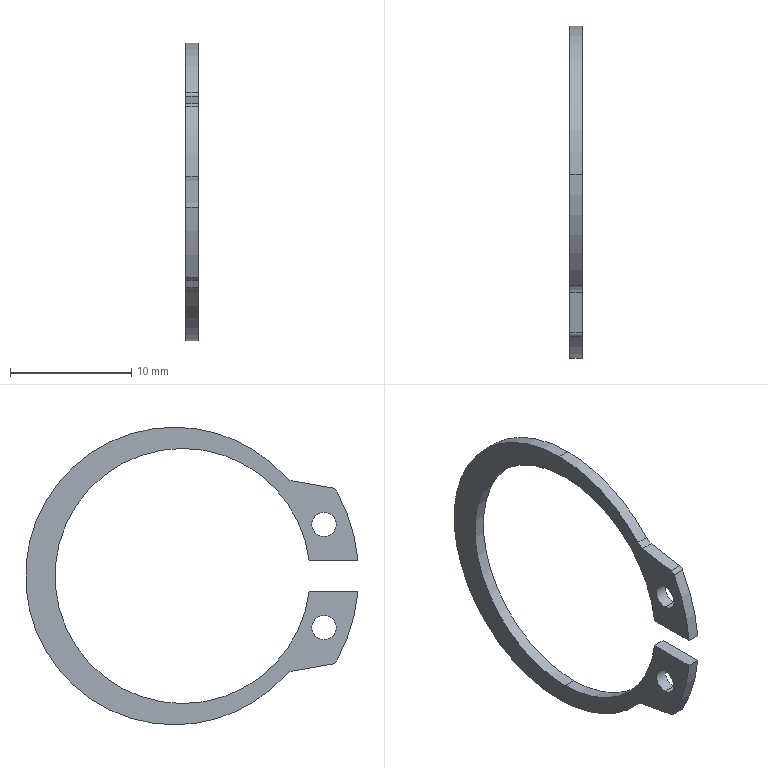Component | SolidWorks | XXXXX08-01-040514RotaryDriveShaft-1_22_T894.1-1 | 1 solid | 22 faces | box 1 x 27.37 x 24.5 mm | volume 155 mm3 | cylinder 16 | plane 6 | commonest cylinder face diameters 2 x6 24.5 x3 21 x3 1 x2 29 x2 | material 65Mn
build123d program:
from build123d import *

# Parameters (mm, degrees)
MATRIX_EXTRUDE_DEPTH      = 0.5
MATRIX_EXTRUDE_DEPTH_BACK = 0.5
SKETCH1_R                 = 1


with BuildPart() as part:
    # Sketch1 → Matrix-Extrude (new, two sides: drawn at the far end of the back side and taken through both)
    with BuildSketch(Plane.XY.offset(-MATRIX_EXTRUDE_DEPTH_BACK)):
        with BuildLine():
            Line((-1.25, -11.095), (-1.25, -15.116))
            ThreePointArc((-1.25, -15.116), (-4.216, -14.544), (-6.999, -13.369))
            ThreePointArc((-6.999, -13.369), (-7.164, -13.222), (-7.25, -13.018))
            Line((-7.25, -13.018), (-7.832, -9.717))
            ThreePointArc((-7.832, -9.717), (-7.943, -9.404), (-8.151, -9.144))
            ThreePointArc((-8.151, -9.144), (0, 12.25), (8.151, -9.144))
            ThreePointArc((8.151, -9.144), (7.943, -9.404), (7.832, -9.717))
            Line((7.832, -9.717), (7.25, -13.018))
            ThreePointArc((7.25, -13.018), (7.164, -13.222), (6.999, -13.369))
            ThreePointArc((6.999, -13.369), (4.216, -14.544), (1.25, -15.116))
            Line((1.25, -15.116), (1.25, -11.095))
            ThreePointArc((1.25, -11.095), (0, 9.83), (-1.25, -11.095))
        make_face()
        with Locations((-4.25, -12.319)):
            Circle(SKETCH1_R, mode=Mode.SUBTRACT)
        with Locations(Location((4.25, -12.319, 0), (0, 0, 180))):
            Circle(SKETCH1_R, mode=Mode.SUBTRACT)
    extrude(amount=MATRIX_EXTRUDE_DEPTH + MATRIX_EXTRUDE_DEPTH_BACK)


solid = part.part

# Placed as in the assembly
solid = solid.moved(Location((-29.2, 0.67, 0), (0, 90, 0)))
STEP:
#1=CARTESIAN_POINT('',(-1.13,-0.4586,-0.128));
#2=VERTEX_POINT('',#1);
#3=CARTESIAN_POINT('',(-1.13,-0.4586,-0.2067));
#4=VERTEX_POINT('',#3);
#5=CARTESIAN_POINT('',(-1.13,-0.4586,-0.1673));
#6=DIRECTION('',(1.,0.,0.));
#7=DIRECTION('',(0.,0.,1.));
#8=AXIS2_PLACEMENT_3D('',#5,#6,#7);
#9=CIRCLE('',#8,0.03937);
#10=EDGE_CURVE('',#2,#4,#9,.T.);
#11=ORIENTED_EDGE('',*,*,#10,.T.);
#12=CARTESIAN_POINT('',(-1.169,-0.4586,-0.2067));
#13=VERTEX_POINT('',#12);
#14=CARTESIAN_POINT('',(-1.13,-0.4586,-0.2067));
#15=DIRECTION('',(-1.,0.,0.));
#16=VECTOR('',#15,39.37);
#17=LINE('',#14,#16);
#18=EDGE_CURVE('',#4,#13,#17,.T.);
#19=ORIENTED_EDGE('',*,*,#18,.T.);
#20=CARTESIAN_POINT('',(-1.169,-0.4586,-0.128));
#21=VERTEX_POINT('',#20);
#22=CARTESIAN_POINT('',(-1.169,-0.4586,-0.1673));
#23=DIRECTION('',(1.,0.,0.));
#24=DIRECTION('',(0.,0.,1.));
#25=AXIS2_PLACEMENT_3D('',#22,#23,#24);
#26=CIRCLE('',#25,0.03937);
#27=EDGE_CURVE('',#21,#13,#26,.T.);
#28=ORIENTED_EDGE('',*,*,#27,.F.);
#29=CARTESIAN_POINT('',(-1.13,-0.4586,-0.128));
#30=DIRECTION('',(-1.,0.,0.));
#31=VECTOR('',#30,39.37);
#32=LINE('',#29,#31);
#33=EDGE_CURVE('',#2,#21,#32,.T.);
#34=ORIENTED_EDGE('',*,*,#33,.F.);
#35=EDGE_LOOP('',(#11,#19,#28,#34));
#36=FACE_OUTER_BOUND('',#35,.T.);
#37=CARTESIAN_POINT('',(-1.13,-0.4586,-0.1673));
#38=DIRECTION('',(-1.,0.,0.));
#39=DIRECTION('',(0.,0.,1.));
#40=AXIS2_PLACEMENT_3D('',#37,#38,#39);
#41=CYLINDRICAL_SURFACE('',#40,0.03937);
#42=ADVANCED_FACE('',(#36),#41,.F.);
#43=CARTESIAN_POINT('',(-1.13,-0.4586,0.2067));
#44=VERTEX_POINT('',#43);
#45=CARTESIAN_POINT('',(-1.13,-0.4586,0.128));
#46=VERTEX_POINT('',#45);
#47=CARTESIAN_POINT('',(-1.13,-0.4586,0.1673));
#48=DIRECTION('',(1.,0.,0.));
#49=DIRECTION('',(0.,0.,-1.));
#50=AXIS2_PLACEMENT_3D('',#47,#48,#49);
#51=CIRCLE('',#50,0.03937);
#52=EDGE_CURVE('',#44,#46,#51,.T.);
#53=ORIENTED_EDGE('',*,*,#52,.T.);
#54=CARTESIAN_POINT('',(-1.169,-0.4586,0.128));
#55=VERTEX_POINT('',#54);
#56=CARTESIAN_POINT('',(-1.13,-0.4586,0.128));
#57=DIRECTION('',(-1.,0.,0.));
#58=VECTOR('',#57,39.37);
#59=LINE('',#56,#58);
#60=EDGE_CURVE('',#46,#55,#59,.T.);
#61=ORIENTED_EDGE('',*,*,#60,.T.);
#62=CARTESIAN_POINT('',(-1.169,-0.4586,0.2067));
#63=VERTEX_POINT('',#62);
#64=CARTESIAN_POINT('',(-1.169,-0.4586,0.1673));
#65=DIRECTION('',(1.,0.,0.));
#66=DIRECTION('',(0.,0.,-1.));
#67=AXIS2_PLACEMENT_3D('',#64,#65,#66);
#68=CIRCLE('',#67,0.03937);
#69=EDGE_CURVE('',#63,#55,#68,.T.);
#70=ORIENTED_EDGE('',*,*,#69,.F.);
#71=CARTESIAN_POINT('',(-1.13,-0.4586,0.2067));
#72=DIRECTION('',(-1.,0.,0.));
#73=VECTOR('',#72,39.37);
#74=LINE('',#71,#73);
#75=EDGE_CURVE('',#44,#63,#74,.T.);
#76=ORIENTED_EDGE('',*,*,#75,.F.);
#77=EDGE_LOOP('',(#53,#61,#70,#76));
#78=FACE_OUTER_BOUND('',#77,.T.);
#79=CARTESIAN_POINT('',(-1.13,-0.4586,0.1673));
#80=DIRECTION('',(-1.,0.,0.));
#81=DIRECTION('',(0.,0.,1.));
#82=AXIS2_PLACEMENT_3D('',#79,#80,#81);
#83=CYLINDRICAL_SURFACE('',#82,0.03937);
#84=ADVANCED_FACE('',(#78),#83,.F.);
#85=CARTESIAN_POINT('',(-1.13,0.02638,-0.4823));
#86=VERTEX_POINT('',#85);
#87=CARTESIAN_POINT('',(-1.13,0.02638,0.4823));
#88=VERTEX_POINT('',#87);
#89=CARTESIAN_POINT('',(-1.13,0.02638,-0.));
#90=DIRECTION('',(1.,0.,0.));
#91=DIRECTION('',(0.,0.,-1.));
#92=AXIS2_PLACEMENT_3D('',#89,#90,#91);
#93=CIRCLE('',#92,0.4823);
#94=EDGE_CURVE('',#86,#88,#93,.T.);
#95=ORIENTED_EDGE('',*,*,#94,.F.);
#96=CARTESIAN_POINT('',(-1.169,0.02638,-0.4823));
#97=VERTEX_POINT('',#96);
#98=CARTESIAN_POINT('',(-1.13,0.02638,-0.4823));
#99=DIRECTION('',(-1.,0.,0.));
#100=VECTOR('',#99,39.37);
#101=LINE('',#98,#100);
#102=EDGE_CURVE('',#86,#97,#101,.T.);
#103=ORIENTED_EDGE('',*,*,#102,.T.);
#104=CARTESIAN_POINT('',(-1.169,0.02638,0.4823));
#105=VERTEX_POINT('',#104);
#106=CARTESIAN_POINT('',(-1.169,0.02638,-0.));
#107=DIRECTION('',(1.,0.,0.));
#108=DIRECTION('',(0.,0.,-1.));
#109=AXIS2_PLACEMENT_3D('',#106,#107,#108);
#110=CIRCLE('',#109,0.4823);
#111=EDGE_CURVE('',#97,#105,#110,.T.);
#112=ORIENTED_EDGE('',*,*,#111,.T.);
#113=CARTESIAN_POINT('',(-1.13,0.02638,0.4823));
#114=DIRECTION('',(-1.,0.,0.));
#115=VECTOR('',#114,39.37);
#116=LINE('',#113,#115);
#117=EDGE_CURVE('',#88,#105,#116,.T.);
#118=ORIENTED_EDGE('',*,*,#117,.F.);
#119=EDGE_LOOP('',(#95,#103,#112,#118));
#120=FACE_OUTER_BOUND('',#119,.T.);
#121=CARTESIAN_POINT('',(-1.13,0.02638,-0.));
#122=DIRECTION('',(-1.,0.,0.));
#123=DIRECTION('',(0.,0.,1.));
#124=AXIS2_PLACEMENT_3D('',#121,#122,#123);
#125=CYLINDRICAL_SURFACE('',#124,0.4823);
#126=ADVANCED_FACE('',(#120),#125,.T.);
#127=CARTESIAN_POINT('',(-1.13,-0.3336,0.3209));
#128=VERTEX_POINT('',#127);
#129=CARTESIAN_POINT('',(-1.13,0.02638,-0.));
#130=DIRECTION('',(1.,0.,0.));
#131=DIRECTION('',(0.,0.,-1.));
#132=AXIS2_PLACEMENT_3D('',#129,#130,#131);
#133=CIRCLE('',#132,0.4823);
#134=EDGE_CURVE('',#88,#128,#133,.T.);
#135=ORIENTED_EDGE('',*,*,#134,.F.);
#136=ORIENTED_EDGE('',*,*,#117,.T.);
#137=CARTESIAN_POINT('',(-1.169,-0.3336,0.3209));
#138=VERTEX_POINT('',#137);
#139=CARTESIAN_POINT('',(-1.169,0.02638,-0.));
#140=DIRECTION('',(1.,0.,0.));
#141=DIRECTION('',(0.,0.,-1.));
#142=AXIS2_PLACEMENT_3D('',#139,#140,#141);
#143=CIRCLE('',#142,0.4823);
#144=EDGE_CURVE('',#105,#138,#143,.T.);
#145=ORIENTED_EDGE('',*,*,#144,.T.);
#146=CARTESIAN_POINT('',(-1.13,-0.3336,0.3209));
#147=DIRECTION('',(-1.,0.,0.));
#148=VECTOR('',#147,39.37);
#149=LINE('',#146,#148);
#150=EDGE_CURVE('',#128,#138,#149,.T.);
#151=ORIENTED_EDGE('',*,*,#150,.F.);
#152=EDGE_LOOP('',(#135,#136,#145,#151));
#153=FACE_OUTER_BOUND('',#152,.T.);
#154=CARTESIAN_POINT('',(-1.13,0.02638,-0.));
#155=DIRECTION('',(-1.,0.,0.));
#156=DIRECTION('',(0.,0.,1.));
#157=AXIS2_PLACEMENT_3D('',#154,#155,#156);
#158=CYLINDRICAL_SURFACE('',#157,0.4823);
#159=ADVANCED_FACE('',(#153),#158,.T.);
#160=CARTESIAN_POINT('',(-1.13,0.,-0.4134));
#161=VERTEX_POINT('',#160);
#162=CARTESIAN_POINT('',(-1.13,-0.4104,-0.04921));
#163=VERTEX_POINT('',#162);
#164=CARTESIAN_POINT('',(-1.13,0.,-0.));
#165=DIRECTION('',(-1.,0.,0.));
#166=DIRECTION('',(0.,0.,-1.));
#167=AXIS2_PLACEMENT_3D('',#164,#165,#166);
#168=CIRCLE('',#167,0.4134);
#169=EDGE_CURVE('',#161,#163,#168,.T.);
#170=ORIENTED_EDGE('',*,*,#169,.F.);
#171=CARTESIAN_POINT('',(-1.169,0.,-0.4134));
#172=VERTEX_POINT('',#171);
#173=CARTESIAN_POINT('',(-1.13,0.,-0.4134));
#174=DIRECTION('',(-1.,0.,0.));
#175=VECTOR('',#174,39.37);
#176=LINE('',#173,#175);
#177=EDGE_CURVE('',#161,#172,#176,.T.);
#178=ORIENTED_EDGE('',*,*,#177,.T.);
#179=CARTESIAN_POINT('',(-1.169,-0.4104,-0.04921));
#180=VERTEX_POINT('',#179);
#181=CARTESIAN_POINT('',(-1.169,0.,-0.));
#182=DIRECTION('',(-1.,0.,0.));
#183=DIRECTION('',(0.,0.,-1.));
#184=AXIS2_PLACEMENT_3D('',#181,#182,#183);
#185=CIRCLE('',#184,0.4134);
#186=EDGE_CURVE('',#172,#180,#185,.T.);
#187=ORIENTED_EDGE('',*,*,#186,.T.);
#188=CARTESIAN_POINT('',(-1.13,-0.4104,-0.04921));
#189=DIRECTION('',(-1.,0.,0.));
#190=VECTOR('',#189,39.37);
#191=LINE('',#188,#190);
#192=EDGE_CURVE('',#163,#180,#191,.T.);
#193=ORIENTED_EDGE('',*,*,#192,.F.);
#194=EDGE_LOOP('',(#170,#178,#187,#193));
#195=FACE_OUTER_BOUND('',#194,.T.);
#196=CARTESIAN_POINT('',(-1.13,0.,-0.));
#197=DIRECTION('',(-1.,0.,0.));
#198=DIRECTION('',(0.,0.,1.));
#199=AXIS2_PLACEMENT_3D('',#196,#197,#198);
#200=CYLINDRICAL_SURFACE('',#199,0.4134);
#201=ADVANCED_FACE('',(#195),#200,.F.);
#202=ORIENTED_EDGE('',*,*,#177,.F.);
#203=CARTESIAN_POINT('',(-1.13,0.,0.4134));
#204=VERTEX_POINT('',#203);
#205=CARTESIAN_POINT('',(-1.13,0.,-0.));
#206=DIRECTION('',(-1.,0.,0.));
#207=DIRECTION('',(0.,0.,-1.));
#208=AXIS2_PLACEMENT_3D('',#205,#206,#207);
#209=CIRCLE('',#208,0.4134);
#210=EDGE_CURVE('',#204,#161,#209,.T.);
#211=ORIENTED_EDGE('',*,*,#210,.F.);
#212=CARTESIAN_POINT('',(-1.169,0.,0.4134));
#213=VERTEX_POINT('',#212);
#214=CARTESIAN_POINT('',(-1.13,0.,0.4134));
#215=DIRECTION('',(-1.,0.,0.));
#216=VECTOR('',#215,39.37);
#217=LINE('',#214,#216);
#218=EDGE_CURVE('',#204,#213,#217,.T.);
#219=ORIENTED_EDGE('',*,*,#218,.T.);
#220=CARTESIAN_POINT('',(-1.169,0.,-0.));
#221=DIRECTION('',(-1.,0.,0.));
#222=DIRECTION('',(0.,0.,-1.));
#223=AXIS2_PLACEMENT_3D('',#220,#221,#222);
#224=CIRCLE('',#223,0.4134);
#225=EDGE_CURVE('',#213,#172,#224,.T.);
#226=ORIENTED_EDGE('',*,*,#225,.T.);
#227=EDGE_LOOP('',(#202,#211,#219,#226));
#228=FACE_OUTER_BOUND('',#227,.T.);
#229=CARTESIAN_POINT('',(-1.13,0.,-0.));
#230=DIRECTION('',(-1.,0.,0.));
#231=DIRECTION('',(0.,0.,1.));
#232=AXIS2_PLACEMENT_3D('',#229,#230,#231);
#233=CYLINDRICAL_SURFACE('',#232,0.4134);
#234=ADVANCED_FACE('',(#228),#233,.F.);
#235=ORIENTED_EDGE('',*,*,#52,.F.);
#236=CARTESIAN_POINT('',(-1.13,-0.4586,0.1673));
#237=DIRECTION('',(1.,0.,0.));
#238=DIRECTION('',(0.,0.,-1.));
#239=AXIS2_PLACEMENT_3D('',#236,#237,#238);
#240=CIRCLE('',#239,0.03937);
#241=EDGE_CURVE('',#46,#44,#240,.T.);
#242=ORIENTED_EDGE('',*,*,#241,.F.);
#243=EDGE_LOOP('',(#235,#242));
#244=FACE_BOUND('',#243,.T.);
#245=CARTESIAN_POINT('',(-1.13,-0.3562,0.3083));
#246=VERTEX_POINT('',#245);
#247=CARTESIAN_POINT('',(-1.13,-0.363,0.3471));
#248=DIRECTION('',(-1.,0.,0.));
#249=DIRECTION('',(0.,0.,-1.));
#250=AXIS2_PLACEMENT_3D('',#247,#248,#249);
#251=CIRCLE('',#250,0.03937);
#252=EDGE_CURVE('',#128,#246,#251,.T.);
#253=ORIENTED_EDGE('',*,*,#252,.T.);
#254=CARTESIAN_POINT('',(-1.13,-0.4861,0.2854));
#255=VERTEX_POINT('',#254);
#256=CARTESIAN_POINT('',(-1.13,-0.3562,0.3083));
#257=DIRECTION('',(0.,-0.9848,-0.1736));
#258=VECTOR('',#257,39.37);
#259=LINE('',#256,#258);
#260=EDGE_CURVE('',#246,#255,#259,.T.);
#261=ORIENTED_EDGE('',*,*,#260,.T.);
#262=CARTESIAN_POINT('',(-1.13,-0.5,0.2755));
#263=VERTEX_POINT('',#262);
#264=CARTESIAN_POINT('',(-1.13,-0.4827,0.266));
#265=DIRECTION('',(1.,0.,0.));
#266=DIRECTION('',(0.,0.,1.));
#267=AXIS2_PLACEMENT_3D('',#264,#265,#266);
#268=CIRCLE('',#267,0.01969);
#269=EDGE_CURVE('',#255,#263,#268,.T.);
#270=ORIENTED_EDGE('',*,*,#269,.T.);
#271=CARTESIAN_POINT('',(-1.13,-0.5687,0.04921));
#272=VERTEX_POINT('',#271);
#273=CARTESIAN_POINT('',(-1.13,0.,-0.));
#274=DIRECTION('',(1.,0.,0.));
#275=DIRECTION('',(0.,0.,1.));
#276=AXIS2_PLACEMENT_3D('',#273,#274,#275);
#277=CIRCLE('',#276,0.5709);
#278=EDGE_CURVE('',#263,#272,#277,.T.);
#279=ORIENTED_EDGE('',*,*,#278,.T.);
#280=CARTESIAN_POINT('',(-1.13,-0.4104,0.04921));
#281=VERTEX_POINT('',#280);
#282=CARTESIAN_POINT('',(-1.13,-0.4104,0.04921));
#283=DIRECTION('',(0.,1.,0.));
#284=VECTOR('',#283,39.37);
#285=LINE('',#282,#284);
#286=EDGE_CURVE('',#272,#281,#285,.T.);
#287=ORIENTED_EDGE('',*,*,#286,.T.);
#288=CARTESIAN_POINT('',(-1.13,0.,-0.));
#289=DIRECTION('',(-1.,0.,0.));
#290=DIRECTION('',(0.,0.,-1.));
#291=AXIS2_PLACEMENT_3D('',#288,#289,#290);
#292=CIRCLE('',#291,0.4134);
#293=EDGE_CURVE('',#281,#204,#292,.T.);
#294=ORIENTED_EDGE('',*,*,#293,.T.);
#295=ORIENTED_EDGE('',*,*,#210,.T.);
#296=ORIENTED_EDGE('',*,*,#169,.T.);
#297=CARTESIAN_POINT('',(-1.13,-0.5687,-0.04921));
#298=VERTEX_POINT('',#297);
#299=CARTESIAN_POINT('',(-1.13,-0.4104,-0.04921));
#300=DIRECTION('',(0.,-1.,-0.));
#301=VECTOR('',#300,39.37);
#302=LINE('',#299,#301);
#303=EDGE_CURVE('',#163,#298,#302,.T.);
#304=ORIENTED_EDGE('',*,*,#303,.T.);
#305=CARTESIAN_POINT('',(-1.13,-0.5,-0.2755));
#306=VERTEX_POINT('',#305);
#307=CARTESIAN_POINT('',(-1.13,0.,-0.));
#308=DIRECTION('',(1.,0.,0.));
#309=DIRECTION('',(0.,0.,-1.));
#310=AXIS2_PLACEMENT_3D('',#307,#308,#309);
#311=CIRCLE('',#310,0.5709);
#312=EDGE_CURVE('',#298,#306,#311,.T.);
#313=ORIENTED_EDGE('',*,*,#312,.T.);
#314=CARTESIAN_POINT('',(-1.13,-0.4861,-0.2854));
#315=VERTEX_POINT('',#314);
#316=CARTESIAN_POINT('',(-1.13,-0.4827,-0.266));
#317=DIRECTION('',(1.,0.,0.));
#318=DIRECTION('',(0.,0.,-1.));
#319=AXIS2_PLACEMENT_3D('',#316,#317,#318);
#320=CIRCLE('',#319,0.01969);
#321=EDGE_CURVE('',#306,#315,#320,.T.);
#322=ORIENTED_EDGE('',*,*,#321,.T.);
#323=CARTESIAN_POINT('',(-1.13,-0.3562,-0.3083));
#324=VERTEX_POINT('',#323);
#325=CARTESIAN_POINT('',(-1.13,-0.3562,-0.3083));
#326=DIRECTION('',(0.,0.9848,-0.1736));
#327=VECTOR('',#326,39.37);
#328=LINE('',#325,#327);
#329=EDGE_CURVE('',#315,#324,#328,.T.);
#330=ORIENTED_EDGE('',*,*,#329,.T.);
#331=CARTESIAN_POINT('',(-1.13,-0.3336,-0.3209));
#332=VERTEX_POINT('',#331);
#333=CARTESIAN_POINT('',(-1.13,-0.363,-0.3471));
#334=DIRECTION('',(-1.,0.,0.));
#335=DIRECTION('',(0.,0.,1.));
#336=AXIS2_PLACEMENT_3D('',#333,#334,#335);
#337=CIRCLE('',#336,0.03937);
#338=EDGE_CURVE('',#324,#332,#337,.T.);
#339=ORIENTED_EDGE('',*,*,#338,.T.);
#340=CARTESIAN_POINT('',(-1.13,0.02638,-0.));
#341=DIRECTION('',(1.,0.,0.));
#342=DIRECTION('',(0.,0.,-1.));
#343=AXIS2_PLACEMENT_3D('',#340,#341,#342);
#344=CIRCLE('',#343,0.4823);
#345=EDGE_CURVE('',#332,#86,#344,.T.);
#346=ORIENTED_EDGE('',*,*,#345,.T.);
#347=ORIENTED_EDGE('',*,*,#94,.T.);
#348=ORIENTED_EDGE('',*,*,#134,.T.);
#349=EDGE_LOOP('',(#253,#261,#270,#279,#287,#294,#295,#296,#304,#313,#322,#330,#339,#346,#347,#348));
#350=FACE_OUTER_BOUND('',#349,.T.);
#351=ORIENTED_EDGE('',*,*,#10,.F.);
#352=CARTESIAN_POINT('',(-1.13,-0.4586,-0.1673));
#353=DIRECTION('',(1.,0.,0.));
#354=DIRECTION('',(0.,0.,1.));
#355=AXIS2_PLACEMENT_3D('',#352,#353,#354);
#356=CIRCLE('',#355,0.03937);
#357=EDGE_CURVE('',#4,#2,#356,.T.);
#358=ORIENTED_EDGE('',*,*,#357,.F.);
#359=EDGE_LOOP('',(#351,#358));
#360=FACE_BOUND('',#359,.T.);
#361=CARTESIAN_POINT('',(-1.13,-0.363,0.3471));
#362=DIRECTION('',(1.,0.,0.));
#363=DIRECTION('',(0.,0.,-1.));
#364=AXIS2_PLACEMENT_3D('',#361,#362,#363);
#365=PLANE('',#364);
#366=ADVANCED_FACE('',(#244,#350,#360),#365,.T.);
#367=ORIENTED_EDGE('',*,*,#150,.T.);
#368=CARTESIAN_POINT('',(-1.169,-0.3562,0.3083));
#369=VERTEX_POINT('',#368);
#370=CARTESIAN_POINT('',(-1.169,-0.363,0.3471));
#371=DIRECTION('',(-1.,0.,0.));
#372=DIRECTION('',(0.,0.,-1.));
#373=AXIS2_PLACEMENT_3D('',#370,#371,#372);
#374=CIRCLE('',#373,0.03937);
#375=EDGE_CURVE('',#138,#369,#374,.T.);
#376=ORIENTED_EDGE('',*,*,#375,.T.);
#377=CARTESIAN_POINT('',(-1.13,-0.3562,0.3083));
#378=DIRECTION('',(-1.,0.,0.));
#379=VECTOR('',#378,39.37);
#380=LINE('',#377,#379);
#381=EDGE_CURVE('',#246,#369,#380,.T.);
#382=ORIENTED_EDGE('',*,*,#381,.F.);
#383=ORIENTED_EDGE('',*,*,#252,.F.);
#384=EDGE_LOOP('',(#367,#376,#382,#383));
#385=FACE_OUTER_BOUND('',#384,.T.);
#386=CARTESIAN_POINT('',(-1.13,-0.363,0.3471));
#387=DIRECTION('',(-1.,0.,0.));
#388=DIRECTION('',(0.,0.,1.));
#389=AXIS2_PLACEMENT_3D('',#386,#387,#388);
#390=CYLINDRICAL_SURFACE('',#389,0.03937);
#391=ADVANCED_FACE('',(#385),#390,.F.);
#392=ORIENTED_EDGE('',*,*,#381,.T.);
#393=CARTESIAN_POINT('',(-1.169,-0.4861,0.2854));
#394=VERTEX_POINT('',#393);
#395=CARTESIAN_POINT('',(-1.169,-0.3562,0.3083));
#396=DIRECTION('',(0.,-0.9848,-0.1736));
#397=VECTOR('',#396,39.37);
#398=LINE('',#395,#397);
#399=EDGE_CURVE('',#369,#394,#398,.T.);
#400=ORIENTED_EDGE('',*,*,#399,.T.);
#401=CARTESIAN_POINT('',(-1.13,-0.4861,0.2854));
#402=DIRECTION('',(-1.,0.,0.));
#403=VECTOR('',#402,39.37);
#404=LINE('',#401,#403);
#405=EDGE_CURVE('',#255,#394,#404,.T.);
#406=ORIENTED_EDGE('',*,*,#405,.F.);
#407=ORIENTED_EDGE('',*,*,#260,.F.);
#408=EDGE_LOOP('',(#392,#400,#406,#407));
#409=FACE_OUTER_BOUND('',#408,.T.);
#410=CARTESIAN_POINT('',(-1.13,-0.3562,0.3083));
#411=DIRECTION('',(0.,0.1736,-0.9848));
#412=DIRECTION('',(0.,0.9848,0.1736));
#413=AXIS2_PLACEMENT_3D('',#410,#411,#412);
#414=PLANE('',#413);
#415=ADVANCED_FACE('',(#409),#414,.F.);
#416=ORIENTED_EDGE('',*,*,#405,.T.);
#417=CARTESIAN_POINT('',(-1.169,-0.5,0.2755));
#418=VERTEX_POINT('',#417);
#419=CARTESIAN_POINT('',(-1.169,-0.4827,0.266));
#420=DIRECTION('',(1.,0.,0.));
#421=DIRECTION('',(0.,0.,1.));
#422=AXIS2_PLACEMENT_3D('',#419,#420,#421);
#423=CIRCLE('',#422,0.01969);
#424=EDGE_CURVE('',#394,#418,#423,.T.);
#425=ORIENTED_EDGE('',*,*,#424,.T.);
#426=CARTESIAN_POINT('',(-1.13,-0.5,0.2755));
#427=DIRECTION('',(-1.,0.,0.));
#428=VECTOR('',#427,39.37);
#429=LINE('',#426,#428);
#430=EDGE_CURVE('',#263,#418,#429,.T.);
#431=ORIENTED_EDGE('',*,*,#430,.F.);
#432=ORIENTED_EDGE('',*,*,#269,.F.);
#433=EDGE_LOOP('',(#416,#425,#431,#432));
#434=FACE_OUTER_BOUND('',#433,.T.);
#435=CARTESIAN_POINT('',(-1.13,-0.4827,0.266));
#436=DIRECTION('',(-1.,0.,0.));
#437=DIRECTION('',(0.,0.,1.));
#438=AXIS2_PLACEMENT_3D('',#435,#436,#437);
#439=CYLINDRICAL_SURFACE('',#438,0.01969);
#440=ADVANCED_FACE('',(#434),#439,.T.);
#441=ORIENTED_EDGE('',*,*,#430,.T.);
#442=CARTESIAN_POINT('',(-1.169,-0.5687,0.04921));
#443=VERTEX_POINT('',#442);
#444=CARTESIAN_POINT('',(-1.169,0.,-0.));
#445=DIRECTION('',(1.,0.,0.));
#446=DIRECTION('',(0.,0.,1.));
#447=AXIS2_PLACEMENT_3D('',#444,#445,#446);
#448=CIRCLE('',#447,0.5709);
#449=EDGE_CURVE('',#418,#443,#448,.T.);
#450=ORIENTED_EDGE('',*,*,#449,.T.);
#451=CARTESIAN_POINT('',(-1.13,-0.5687,0.04921));
#452=DIRECTION('',(-1.,0.,0.));
#453=VECTOR('',#452,39.37);
#454=LINE('',#451,#453);
#455=EDGE_CURVE('',#272,#443,#454,.T.);
#456=ORIENTED_EDGE('',*,*,#455,.F.);
#457=ORIENTED_EDGE('',*,*,#278,.F.);
#458=EDGE_LOOP('',(#441,#450,#456,#457));
#459=FACE_OUTER_BOUND('',#458,.T.);
#460=CARTESIAN_POINT('',(-1.13,0.,-0.));
#461=DIRECTION('',(-1.,0.,0.));
#462=DIRECTION('',(0.,0.,1.));
#463=AXIS2_PLACEMENT_3D('',#460,#461,#462);
#464=CYLINDRICAL_SURFACE('',#463,0.5709);
#465=ADVANCED_FACE('',(#459),#464,.T.);
#466=ORIENTED_EDGE('',*,*,#455,.T.);
#467=CARTESIAN_POINT('',(-1.169,-0.4104,0.04921));
#468=VERTEX_POINT('',#467);
#469=CARTESIAN_POINT('',(-1.169,-0.4104,0.04921));
#470=DIRECTION('',(0.,1.,0.));
#471=VECTOR('',#470,39.37);
#472=LINE('',#469,#471);
#473=EDGE_CURVE('',#443,#468,#472,.T.);
#474=ORIENTED_EDGE('',*,*,#473,.T.);
#475=CARTESIAN_POINT('',(-1.13,-0.4104,0.04921));
#476=DIRECTION('',(-1.,0.,0.));
#477=VECTOR('',#476,39.37);
#478=LINE('',#475,#477);
#479=EDGE_CURVE('',#281,#468,#478,.T.);
#480=ORIENTED_EDGE('',*,*,#479,.F.);
#481=ORIENTED_EDGE('',*,*,#286,.F.);
#482=EDGE_LOOP('',(#466,#474,#480,#481));
#483=FACE_OUTER_BOUND('',#482,.T.);
#484=CARTESIAN_POINT('',(-1.13,-0.4104,0.04921));
#485=DIRECTION('',(0.,-0.,1.));
#486=DIRECTION('',(0.,-1.,-0.));
#487=AXIS2_PLACEMENT_3D('',#484,#485,#486);
#488=PLANE('',#487);
#489=ADVANCED_FACE('',(#483),#488,.F.);
#490=ORIENTED_EDGE('',*,*,#218,.F.);
#491=ORIENTED_EDGE('',*,*,#293,.F.);
#492=ORIENTED_EDGE('',*,*,#479,.T.);
#493=CARTESIAN_POINT('',(-1.169,0.,-0.));
#494=DIRECTION('',(-1.,0.,0.));
#495=DIRECTION('',(0.,0.,-1.));
#496=AXIS2_PLACEMENT_3D('',#493,#494,#495);
#497=CIRCLE('',#496,0.4134);
#498=EDGE_CURVE('',#468,#213,#497,.T.);
#499=ORIENTED_EDGE('',*,*,#498,.T.);
#500=EDGE_LOOP('',(#490,#491,#492,#499));
#501=FACE_OUTER_BOUND('',#500,.T.);
#502=CARTESIAN_POINT('',(-1.13,0.,-0.));
#503=DIRECTION('',(-1.,0.,0.));
#504=DIRECTION('',(0.,0.,1.));
#505=AXIS2_PLACEMENT_3D('',#502,#503,#504);
#506=CYLINDRICAL_SURFACE('',#505,0.4134);
#507=ADVANCED_FACE('',(#501),#506,.F.);
#508=ORIENTED_EDGE('',*,*,#192,.T.);
#509=CARTESIAN_POINT('',(-1.169,-0.5687,-0.04921));
#510=VERTEX_POINT('',#509);
#511=CARTESIAN_POINT('',(-1.169,-0.4104,-0.04921));
#512=DIRECTION('',(0.,-1.,-0.));
#513=VECTOR('',#512,39.37);
#514=LINE('',#511,#513);
#515=EDGE_CURVE('',#180,#510,#514,.T.);
#516=ORIENTED_EDGE('',*,*,#515,.T.);
#517=CARTESIAN_POINT('',(-1.13,-0.5687,-0.04921));
#518=DIRECTION('',(-1.,0.,0.));
#519=VECTOR('',#518,39.37);
#520=LINE('',#517,#519);
#521=EDGE_CURVE('',#298,#510,#520,.T.);
#522=ORIENTED_EDGE('',*,*,#521,.F.);
#523=ORIENTED_EDGE('',*,*,#303,.F.);
#524=EDGE_LOOP('',(#508,#516,#522,#523));
#525=FACE_OUTER_BOUND('',#524,.T.);
#526=CARTESIAN_POINT('',(-1.13,-0.4104,-0.04921));
#527=DIRECTION('',(0.,0.,-1.));
#528=DIRECTION('',(0.,1.,0.));
#529=AXIS2_PLACEMENT_3D('',#526,#527,#528);
#530=PLANE('',#529);
#531=ADVANCED_FACE('',(#525),#530,.F.);
#532=ORIENTED_EDGE('',*,*,#521,.T.);
#533=CARTESIAN_POINT('',(-1.169,-0.5,-0.2755));
#534=VERTEX_POINT('',#533);
#535=CARTESIAN_POINT('',(-1.169,0.,-0.));
#536=DIRECTION('',(1.,0.,0.));
#537=DIRECTION('',(0.,0.,-1.));
#538=AXIS2_PLACEMENT_3D('',#535,#536,#537);
#539=CIRCLE('',#538,0.5709);
#540=EDGE_CURVE('',#510,#534,#539,.T.);
#541=ORIENTED_EDGE('',*,*,#540,.T.);
#542=CARTESIAN_POINT('',(-1.13,-0.5,-0.2755));
#543=DIRECTION('',(-1.,0.,0.));
#544=VECTOR('',#543,39.37);
#545=LINE('',#542,#544);
#546=EDGE_CURVE('',#306,#534,#545,.T.);
#547=ORIENTED_EDGE('',*,*,#546,.F.);
#548=ORIENTED_EDGE('',*,*,#312,.F.);
#549=EDGE_LOOP('',(#532,#541,#547,#548));
#550=FACE_OUTER_BOUND('',#549,.T.);
#551=CARTESIAN_POINT('',(-1.13,0.,-0.));
#552=DIRECTION('',(-1.,0.,0.));
#553=DIRECTION('',(0.,0.,1.));
#554=AXIS2_PLACEMENT_3D('',#551,#552,#553);
#555=CYLINDRICAL_SURFACE('',#554,0.5709);
#556=ADVANCED_FACE('',(#550),#555,.T.);
#557=ORIENTED_EDGE('',*,*,#546,.T.);
#558=CARTESIAN_POINT('',(-1.169,-0.4861,-0.2854));
#559=VERTEX_POINT('',#558);
#560=CARTESIAN_POINT('',(-1.169,-0.4827,-0.266));
#561=DIRECTION('',(1.,0.,0.));
#562=DIRECTION('',(0.,0.,-1.));
#563=AXIS2_PLACEMENT_3D('',#560,#561,#562);
#564=CIRCLE('',#563,0.01969);
#565=EDGE_CURVE('',#534,#559,#564,.T.);
#566=ORIENTED_EDGE('',*,*,#565,.T.);
#567=CARTESIAN_POINT('',(-1.13,-0.4861,-0.2854));
#568=DIRECTION('',(-1.,0.,0.));
#569=VECTOR('',#568,39.37);
#570=LINE('',#567,#569);
#571=EDGE_CURVE('',#315,#559,#570,.T.);
#572=ORIENTED_EDGE('',*,*,#571,.F.);
#573=ORIENTED_EDGE('',*,*,#321,.F.);
#574=EDGE_LOOP('',(#557,#566,#572,#573));
#575=FACE_OUTER_BOUND('',#574,.T.);
#576=CARTESIAN_POINT('',(-1.13,-0.4827,-0.266));
#577=DIRECTION('',(-1.,0.,0.));
#578=DIRECTION('',(0.,0.,1.));
#579=AXIS2_PLACEMENT_3D('',#576,#577,#578);
#580=CYLINDRICAL_SURFACE('',#579,0.01969);
#581=ADVANCED_FACE('',(#575),#580,.T.);
#582=ORIENTED_EDGE('',*,*,#571,.T.);
#583=CARTESIAN_POINT('',(-1.169,-0.3562,-0.3083));
#584=VERTEX_POINT('',#583);
#585=CARTESIAN_POINT('',(-1.169,-0.3562,-0.3083));
#586=DIRECTION('',(0.,0.9848,-0.1736));
#587=VECTOR('',#586,39.37);
#588=LINE('',#585,#587);
#589=EDGE_CURVE('',#559,#584,#588,.T.);
#590=ORIENTED_EDGE('',*,*,#589,.T.);
#591=CARTESIAN_POINT('',(-1.13,-0.3562,-0.3083));
#592=DIRECTION('',(-1.,0.,0.));
#593=VECTOR('',#592,39.37);
#594=LINE('',#591,#593);
#595=EDGE_CURVE('',#324,#584,#594,.T.);
#596=ORIENTED_EDGE('',*,*,#595,.F.);
#597=ORIENTED_EDGE('',*,*,#329,.F.);
#598=EDGE_LOOP('',(#582,#590,#596,#597));
#599=FACE_OUTER_BOUND('',#598,.T.);
#600=CARTESIAN_POINT('',(-1.13,-0.3562,-0.3083));
#601=DIRECTION('',(0.,0.1736,0.9848));
#602=DIRECTION('',(0.,-0.9848,0.1736));
#603=AXIS2_PLACEMENT_3D('',#600,#601,#602);
#604=PLANE('',#603);
#605=ADVANCED_FACE('',(#599),#604,.F.);
#606=ORIENTED_EDGE('',*,*,#595,.T.);
#607=CARTESIAN_POINT('',(-1.169,-0.3336,-0.3209));
#608=VERTEX_POINT('',#607);
#609=CARTESIAN_POINT('',(-1.169,-0.363,-0.3471));
#610=DIRECTION('',(-1.,0.,0.));
#611=DIRECTION('',(0.,0.,1.));
#612=AXIS2_PLACEMENT_3D('',#609,#610,#611);
#613=CIRCLE('',#612,0.03937);
#614=EDGE_CURVE('',#584,#608,#613,.T.);
#615=ORIENTED_EDGE('',*,*,#614,.T.);
#616=CARTESIAN_POINT('',(-1.13,-0.3336,-0.3209));
#617=DIRECTION('',(-1.,0.,0.));
#618=VECTOR('',#617,39.37);
#619=LINE('',#616,#618);
#620=EDGE_CURVE('',#332,#608,#619,.T.);
#621=ORIENTED_EDGE('',*,*,#620,.F.);
#622=ORIENTED_EDGE('',*,*,#338,.F.);
#623=EDGE_LOOP('',(#606,#615,#621,#622));
#624=FACE_OUTER_BOUND('',#623,.T.);
#625=CARTESIAN_POINT('',(-1.13,-0.363,-0.3471));
#626=DIRECTION('',(-1.,0.,0.));
#627=DIRECTION('',(0.,0.,1.));
#628=AXIS2_PLACEMENT_3D('',#625,#626,#627);
#629=CYLINDRICAL_SURFACE('',#628,0.03937);
#630=ADVANCED_FACE('',(#624),#629,.F.);
#631=ORIENTED_EDGE('',*,*,#102,.F.);
#632=ORIENTED_EDGE('',*,*,#345,.F.);
#633=ORIENTED_EDGE('',*,*,#620,.T.);
#634=CARTESIAN_POINT('',(-1.169,0.02638,-0.));
#635=DIRECTION('',(1.,0.,0.));
#636=DIRECTION('',(0.,0.,-1.));
#637=AXIS2_PLACEMENT_3D('',#634,#635,#636);
#638=CIRCLE('',#637,0.4823);
#639=EDGE_CURVE('',#608,#97,#638,.T.);
#640=ORIENTED_EDGE('',*,*,#639,.T.);
#641=EDGE_LOOP('',(#631,#632,#633,#640));
#642=FACE_OUTER_BOUND('',#641,.T.);
#643=CARTESIAN_POINT('',(-1.13,0.02638,-0.));
#644=DIRECTION('',(-1.,0.,0.));
#645=DIRECTION('',(0.,0.,1.));
#646=AXIS2_PLACEMENT_3D('',#643,#644,#645);
#647=CYLINDRICAL_SURFACE('',#646,0.4823);
#648=ADVANCED_FACE('',(#642),#647,.T.);
#649=ORIENTED_EDGE('',*,*,#60,.F.);
#650=ORIENTED_EDGE('',*,*,#241,.T.);
#651=ORIENTED_EDGE('',*,*,#75,.T.);
#652=CARTESIAN_POINT('',(-1.169,-0.4586,0.1673));
#653=DIRECTION('',(1.,0.,0.));
#654=DIRECTION('',(0.,0.,-1.));
#655=AXIS2_PLACEMENT_3D('',#652,#653,#654);
#656=CIRCLE('',#655,0.03937);
#657=EDGE_CURVE('',#55,#63,#656,.T.);
#658=ORIENTED_EDGE('',*,*,#657,.F.);
#659=EDGE_LOOP('',(#649,#650,#651,#658));
#660=FACE_OUTER_BOUND('',#659,.T.);
#661=CARTESIAN_POINT('',(-1.13,-0.4586,0.1673));
#662=DIRECTION('',(-1.,0.,0.));
#663=DIRECTION('',(0.,0.,1.));
#664=AXIS2_PLACEMENT_3D('',#661,#662,#663);
#665=CYLINDRICAL_SURFACE('',#664,0.03937);
#666=ADVANCED_FACE('',(#660),#665,.F.);
#667=ORIENTED_EDGE('',*,*,#18,.F.);
#668=ORIENTED_EDGE('',*,*,#357,.T.);
#669=ORIENTED_EDGE('',*,*,#33,.T.);
#670=CARTESIAN_POINT('',(-1.169,-0.4586,-0.1673));
#671=DIRECTION('',(1.,0.,0.));
#672=DIRECTION('',(0.,0.,1.));
#673=AXIS2_PLACEMENT_3D('',#670,#671,#672);
#674=CIRCLE('',#673,0.03937);
#675=EDGE_CURVE('',#13,#21,#674,.T.);
#676=ORIENTED_EDGE('',*,*,#675,.F.);
#677=EDGE_LOOP('',(#667,#668,#669,#676));
#678=FACE_OUTER_BOUND('',#677,.T.);
#679=CARTESIAN_POINT('',(-1.13,-0.4586,-0.1673));
#680=DIRECTION('',(-1.,0.,0.));
#681=DIRECTION('',(0.,0.,1.));
#682=AXIS2_PLACEMENT_3D('',#679,#680,#681);
#683=CYLINDRICAL_SURFACE('',#682,0.03937);
#684=ADVANCED_FACE('',(#678),#683,.F.);
#685=ORIENTED_EDGE('',*,*,#27,.T.);
#686=ORIENTED_EDGE('',*,*,#675,.T.);
#687=EDGE_LOOP('',(#685,#686));
#688=FACE_BOUND('',#687,.T.);
#689=ORIENTED_EDGE('',*,*,#69,.T.);
#690=ORIENTED_EDGE('',*,*,#657,.T.);
#691=EDGE_LOOP('',(#689,#690));
#692=FACE_BOUND('',#691,.T.);
#693=ORIENTED_EDGE('',*,*,#375,.F.);
#694=ORIENTED_EDGE('',*,*,#144,.F.);
#695=ORIENTED_EDGE('',*,*,#111,.F.);
#696=ORIENTED_EDGE('',*,*,#639,.F.);
#697=ORIENTED_EDGE('',*,*,#614,.F.);
#698=ORIENTED_EDGE('',*,*,#589,.F.);
#699=ORIENTED_EDGE('',*,*,#565,.F.);
#700=ORIENTED_EDGE('',*,*,#540,.F.);
#701=ORIENTED_EDGE('',*,*,#515,.F.);
#702=ORIENTED_EDGE('',*,*,#186,.F.);
#703=ORIENTED_EDGE('',*,*,#225,.F.);
#704=ORIENTED_EDGE('',*,*,#498,.F.);
#705=ORIENTED_EDGE('',*,*,#473,.F.);
#706=ORIENTED_EDGE('',*,*,#449,.F.);
#707=ORIENTED_EDGE('',*,*,#424,.F.);
#708=ORIENTED_EDGE('',*,*,#399,.F.);
#709=EDGE_LOOP('',(#693,#694,#695,#696,#697,#698,#699,#700,#701,#702,#703,#704,#705,#706,#707,#708));
#710=FACE_OUTER_BOUND('',#709,.T.);
#711=CARTESIAN_POINT('',(-1.169,-0.363,0.3471));
#712=DIRECTION('',(1.,0.,0.));
#713=DIRECTION('',(0.,0.,-1.));
#714=AXIS2_PLACEMENT_3D('',#711,#712,#713);
#715=PLANE('',#714);
#716=ADVANCED_FACE('',(#688,#692,#710),#715,.F.);
#717=CLOSED_SHELL('',(#42,#84,#126,#159,#201,#234,#366,#391,#415,#440,#465,#489,#507,#531,#556,#581,#605,#630,#648,#666,#684,#716));
#718=MANIFOLD_SOLID_BREP('',#717);
#719=CARTESIAN_POINT('',(0.,0.,0.));
#720=DIRECTION('',(0.,0.,1.));
#721=DIRECTION('',(1.,0.,0.));
#722=AXIS2_PLACEMENT_3D('',#719,#720,#721);
#723=(LENGTH_UNIT()NAMED_UNIT(*)SI_UNIT($,.METRE.));
#724=LENGTH_MEASURE_WITH_UNIT(LENGTH_MEASURE(0.0254),#723);
#725=DIMENSIONAL_EXPONENTS(1.,0.,0.,0.,0.,0.,0.);
#726=(CONVERSION_BASED_UNIT('',#724)LENGTH_UNIT()NAMED_UNIT(#725));
#727=UNCERTAINTY_MEASURE_WITH_UNIT(LENGTH_MEASURE(0.00001),#726,'','');
#728=(NAMED_UNIT(*)PLANE_ANGLE_UNIT()SI_UNIT($,.RADIAN.));
#729=(NAMED_UNIT(*)SI_UNIT($,.STERADIAN.)SOLID_ANGLE_UNIT());
#730=(GEOMETRIC_REPRESENTATION_CONTEXT(3)GLOBAL_UNCERTAINTY_ASSIGNED_CONTEXT((#727))GLOBAL_UNIT_ASSIGNED_CONTEXT((#726,#728,#729))REPRESENTATION_CONTEXT('',''));
#731=ADVANCED_BREP_SHAPE_REPRESENTATION('',(#718,#722),#730);
#732=COLOUR_RGB('',0.7922,0.8196,0.9333);
#733=FILL_AREA_STYLE_COLOUR('',#732);
#734=FILL_AREA_STYLE('',(#733));
#735=SURFACE_STYLE_FILL_AREA(#734);
#736=SURFACE_SIDE_STYLE('',(#735));
#737=SURFACE_STYLE_USAGE(.BOTH.,#736);
#738=PRESENTATION_STYLE_ASSIGNMENT((#737));
#739=STYLED_ITEM('',(#738),#718);
#740=PRESENTATION_LAYER_ASSIGNMENT('','',(#739));
#741=(LENGTH_UNIT()NAMED_UNIT(*)SI_UNIT($,.METRE.));
#742=LENGTH_MEASURE_WITH_UNIT(LENGTH_MEASURE(0.0254),#741);
#743=DIMENSIONAL_EXPONENTS(1.,0.,0.,0.,0.,0.,0.);
#744=(CONVERSION_BASED_UNIT('',#742)LENGTH_UNIT()NAMED_UNIT(#743));
#745=UNCERTAINTY_MEASURE_WITH_UNIT(LENGTH_MEASURE(0.00001),#744,'','');
#746=(NAMED_UNIT(*)PLANE_ANGLE_UNIT()SI_UNIT($,.RADIAN.));
#747=(NAMED_UNIT(*)SI_UNIT($,.STERADIAN.)SOLID_ANGLE_UNIT());
#748=(GEOMETRIC_REPRESENTATION_CONTEXT(3)GLOBAL_UNCERTAINTY_ASSIGNED_CONTEXT((#745))GLOBAL_UNIT_ASSIGNED_CONTEXT((#744,#746,#747))REPRESENTATION_CONTEXT('',''));
#749=MECHANICAL_DESIGN_GEOMETRIC_PRESENTATION_REPRESENTATION('',(#739),#748);